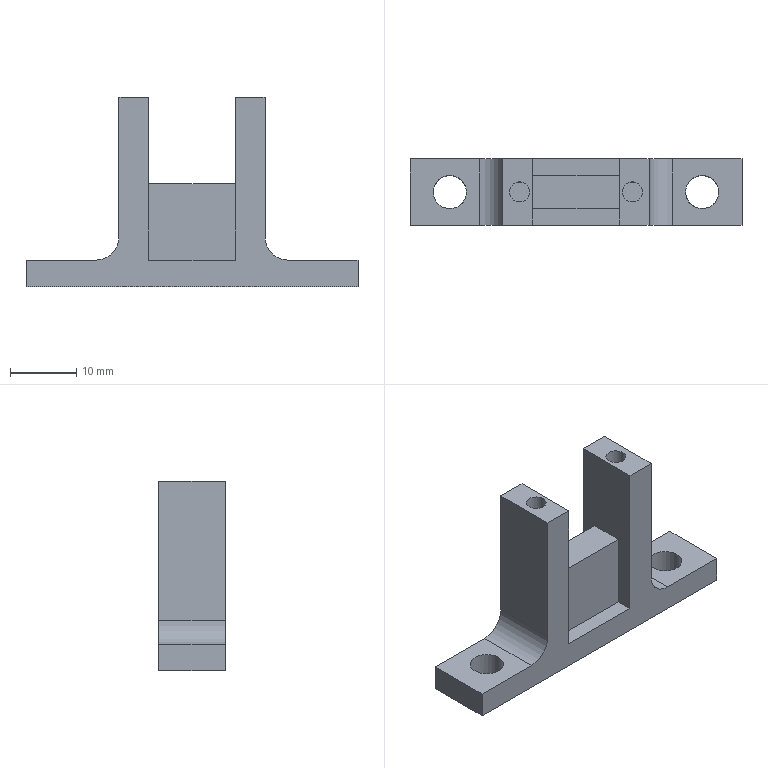Component | NX | UPRIGHT_FRAME | 1 solid | 26 faces | volume 4697 mm3 | plane 20 | cylinder 6 | commonest cylinder face diameters 7 x2 5 x2 3 x2